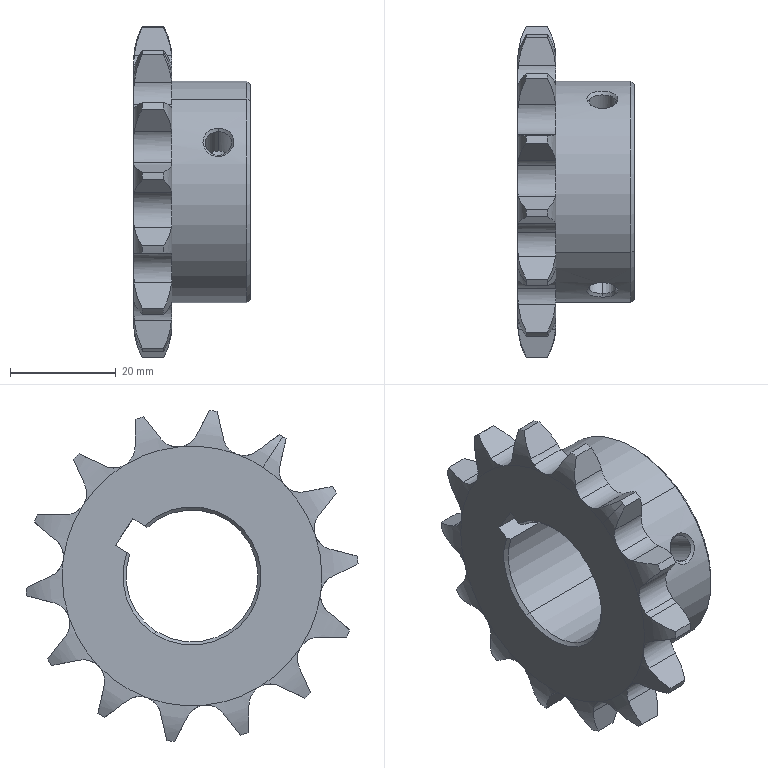Component | SolidWorks | CCD09DriveSprocket-1 | 1 solid | 118 faces | volume 25411 mm3 | cylinder 42 | spline 34 | plane 34 | cone 8 | commonest cylinder face diameters 8.04 x18 63 x15 5 x4 25 x3 42 x2